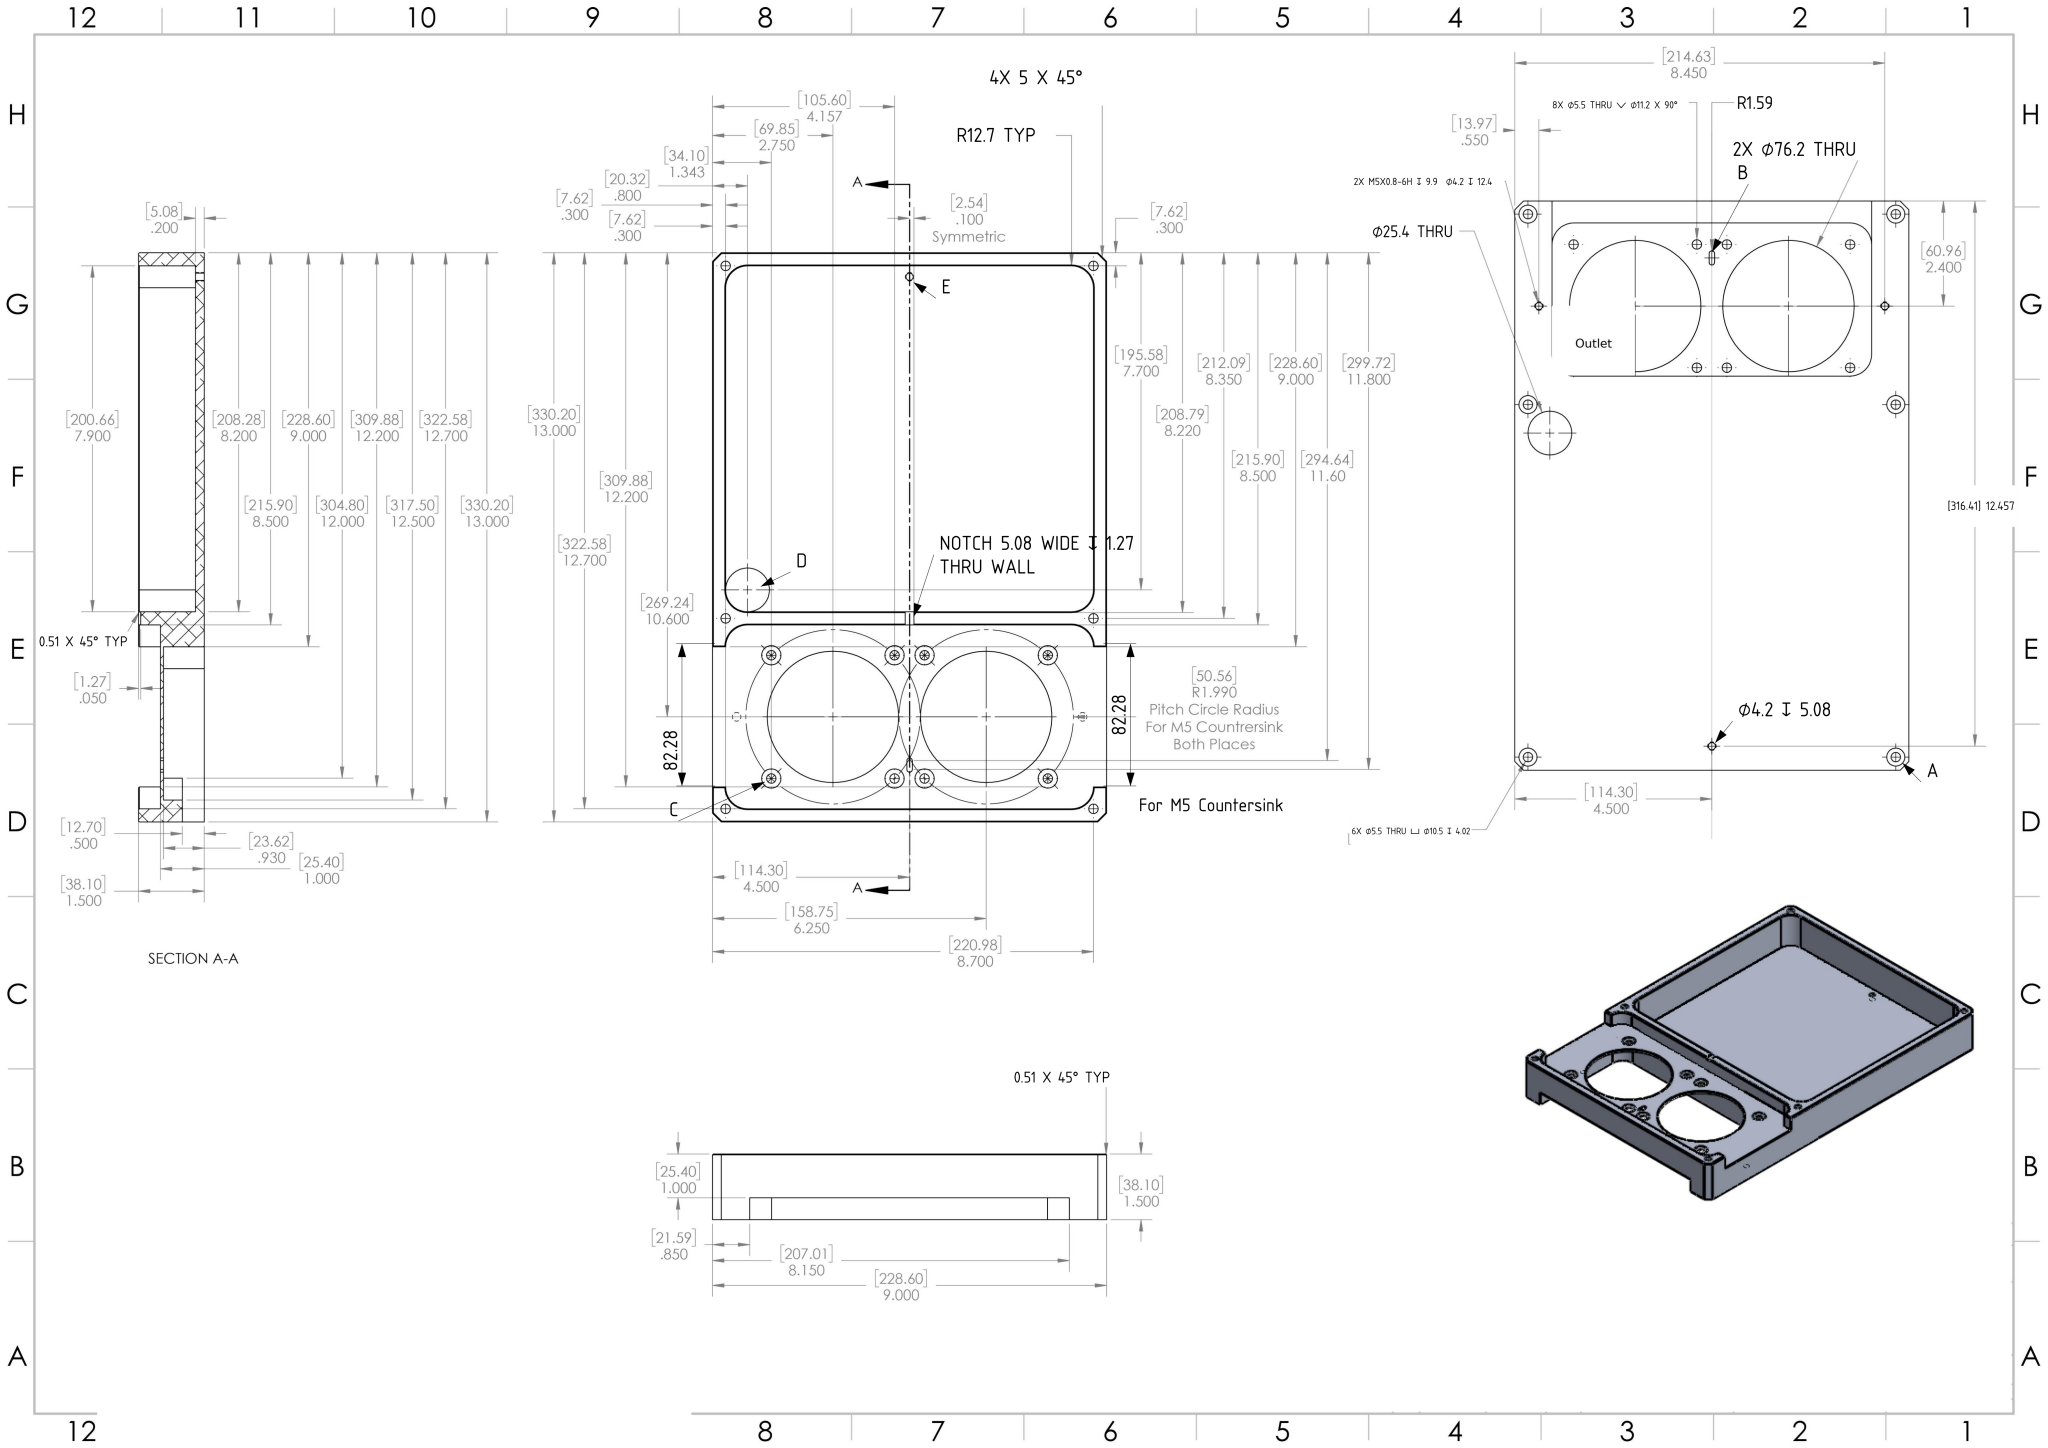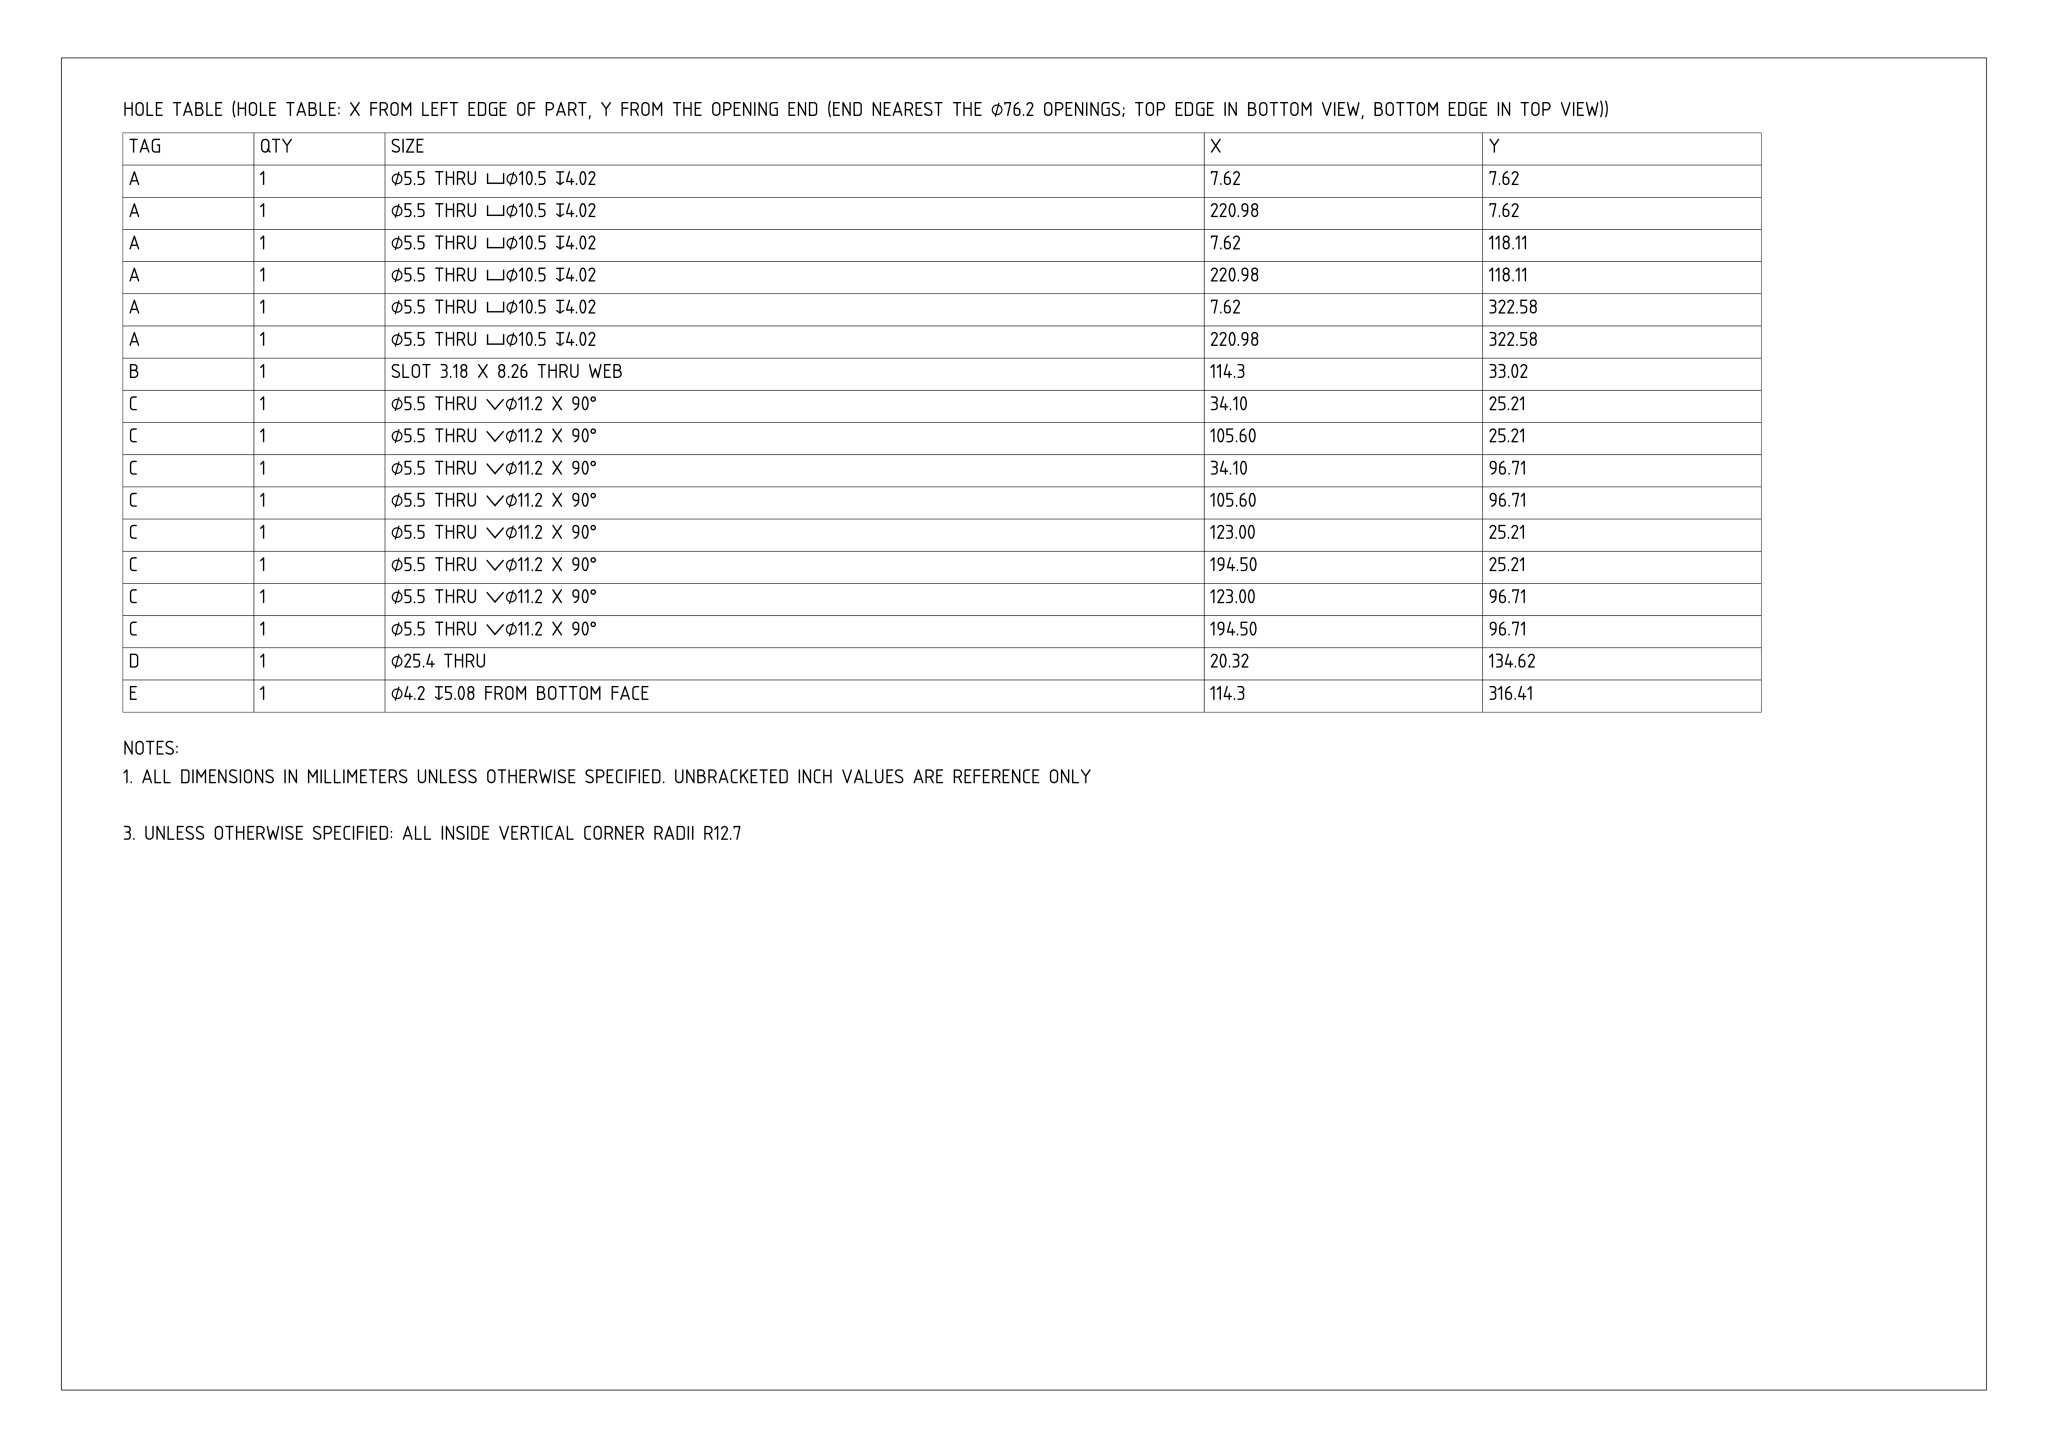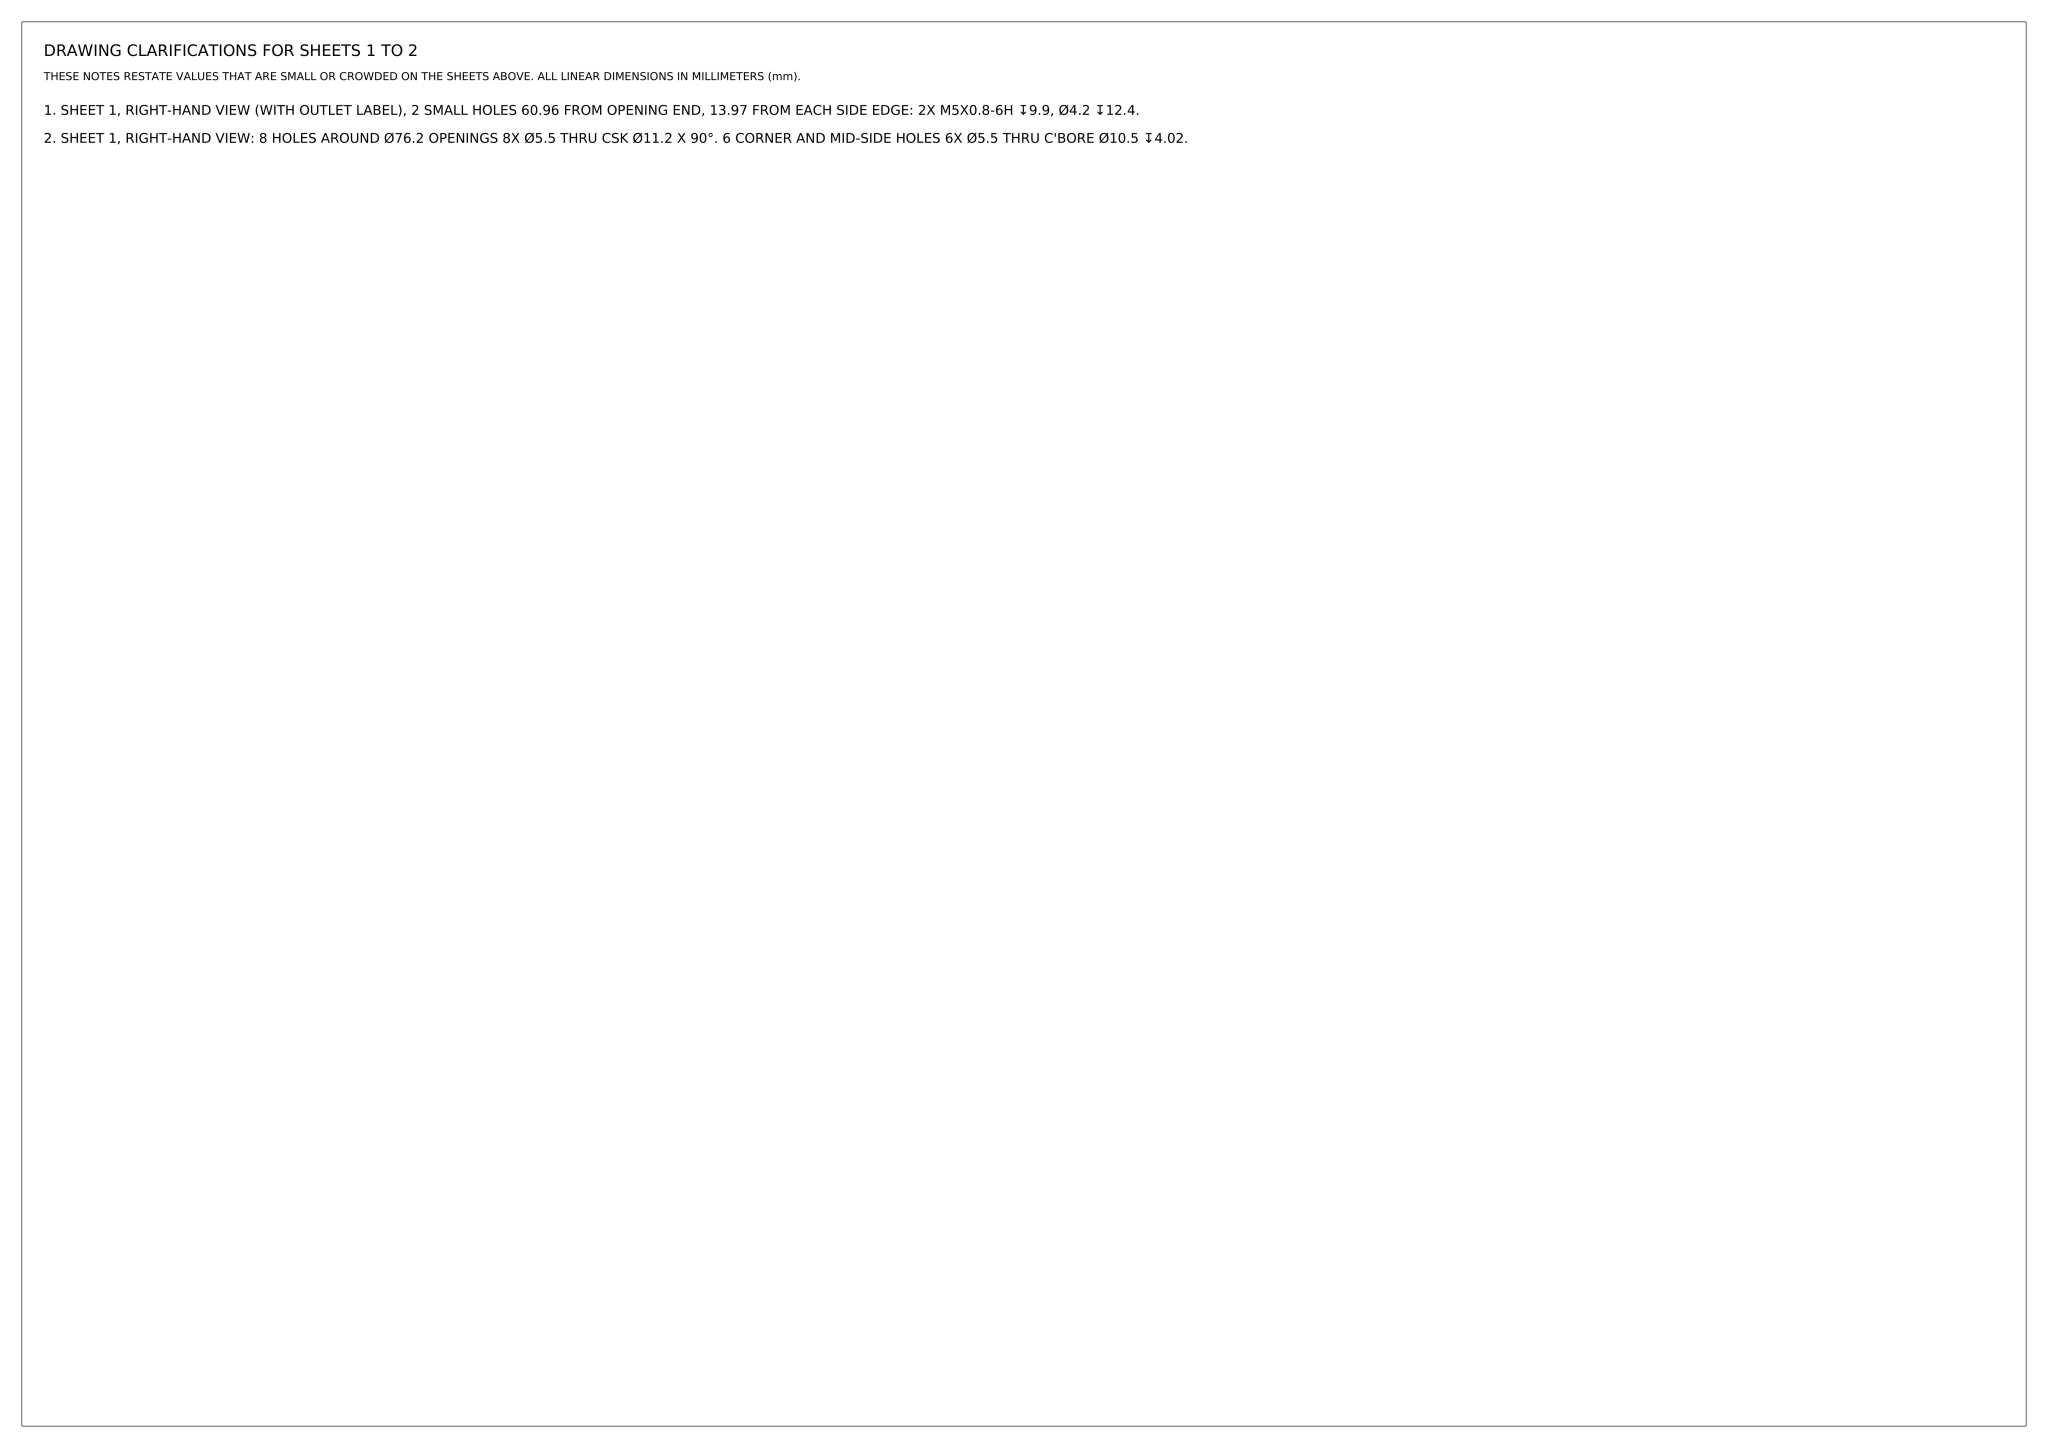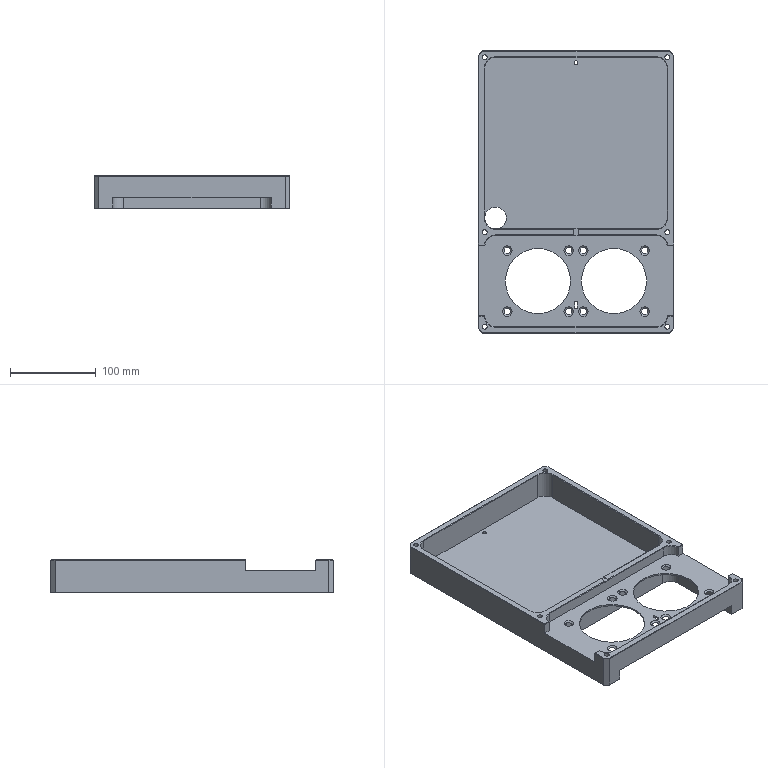Part | NX | mm | 1 solid | 111 faces | box 228.6 x 330.2 x 38.1 mm | volume 717309 mm3 | plane 62 | cylinder 31 | cone 18 | commonest cylinder face diameters 25.4 x12 5.5 x6 10.5 x6 4.2 x3 76.2 x2 3.175 x2